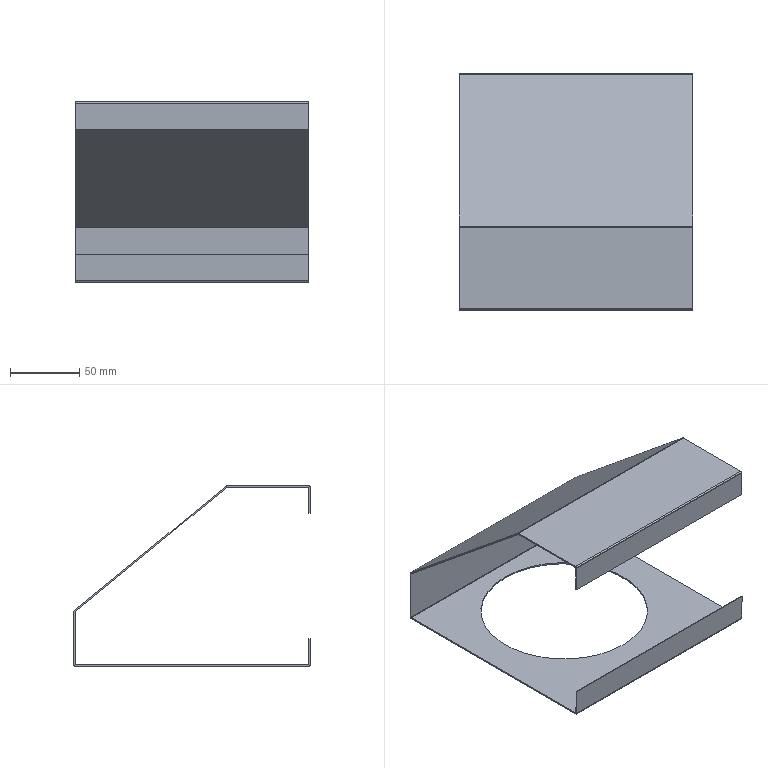Component | SolidWorks | WeldmentDrawing-1_AirDuct1-1 | 1 solid | 48 faces | volume 63865 mm3 | plane 36 | cylinder 12 | commonest cylinder face diameters 2.2 x5 0.2 x5 120 x2